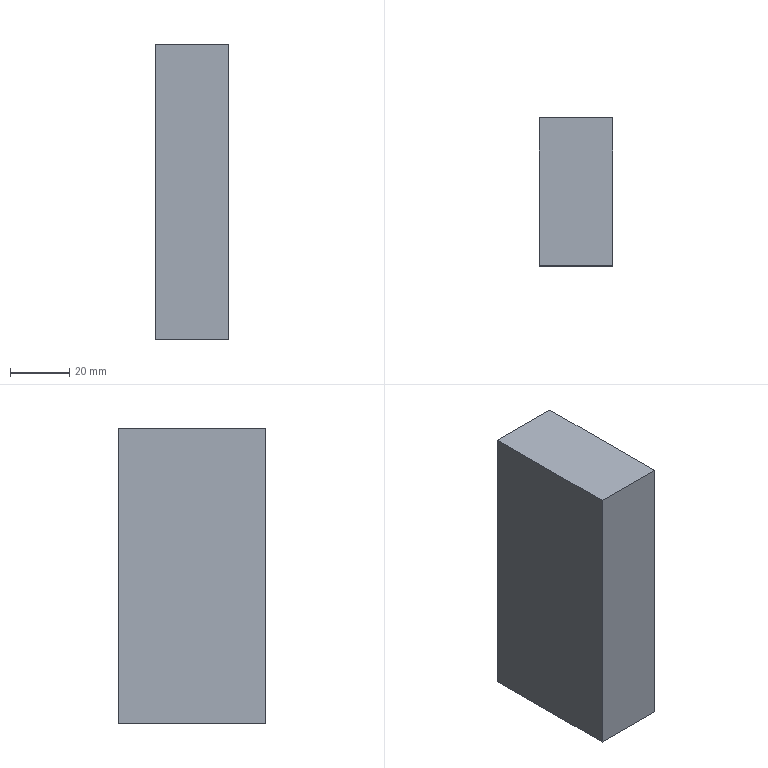Component | NX | SIDE | 1 solid | 6 faces | box 25 x 50 x 100 mm | volume 125000 mm3 | plane 6
STEP:
#1=CARTESIAN_POINT('',(0.,0.,0.));
#2=DIRECTION('',(0.,0.,1.));
#3=DIRECTION('',(1.,0.,0.));
#4=AXIS2_PLACEMENT_3D('',#1,#2,#3);
#5=CARTESIAN_POINT('',(530.662,30.,80.));
#6=VERTEX_POINT('',#5);
#7=CARTESIAN_POINT('',(530.662,30.,-20.));
#8=VERTEX_POINT('',#7);
#9=CARTESIAN_POINT('',(530.662,30.,80.));
#10=DIRECTION('',(0.,-0.,-1.));
#11=VECTOR('',#10,1.);
#12=LINE('',#9,#11);
#13=CARTESIAN_POINT('',(505.662,30.,80.));
#14=DIRECTION('',(0.,-1.,0.));
#15=DIRECTION('',(0.,-0.,-1.));
#16=AXIS2_PLACEMENT_3D('',#13,#14,#15);
#17=PLANE('',#16);
#18=CARTESIAN_POINT('',(0.,25.));
#19=DIRECTION('',(1.,0.));
#20=VECTOR('',#19,1.);
#21=LINE('',#18,#20);
#22=(GEOMETRIC_REPRESENTATION_CONTEXT(2)PARAMETRIC_REPRESENTATION_CONTEXT()REPRESENTATION_CONTEXT('',''));
#23=DEFINITIONAL_REPRESENTATION('',(#21),#22);
#24=PCURVE('',#17,#23);
#25=CARTESIAN_POINT('',(530.662,30.,-20.));
#26=DIRECTION('',(-1.,0.,0.));
#27=DIRECTION('',(0.,0.,-1.));
#28=AXIS2_PLACEMENT_3D('',#25,#26,#27);
#29=PLANE('',#28);
#30=CARTESIAN_POINT('',(-100.,0.));
#31=DIRECTION('',(1.,0.));
#32=VECTOR('',#31,1.);
#33=LINE('',#30,#32);
#34=(GEOMETRIC_REPRESENTATION_CONTEXT(2)PARAMETRIC_REPRESENTATION_CONTEXT()REPRESENTATION_CONTEXT('',''));
#35=DEFINITIONAL_REPRESENTATION('',(#33),#34);
#36=PCURVE('',#29,#35);
#37=SURFACE_CURVE('',#12,(#24,#36),.PCURVE_S1.);
#38=EDGE_CURVE('',#6,#8,#37,.T.);
#39=ORIENTED_EDGE('',*,*,#38,.T.);
#40=CARTESIAN_POINT('',(505.662,30.,-20.));
#41=VERTEX_POINT('',#40);
#42=CARTESIAN_POINT('',(505.662,30.,-20.));
#43=DIRECTION('',(1.,0.,0.));
#44=VECTOR('',#43,1.);
#45=LINE('',#42,#44);
#46=CARTESIAN_POINT('',(100.,0.));
#47=DIRECTION('',(0.,1.));
#48=VECTOR('',#47,1.);
#49=LINE('',#46,#48);
#50=(GEOMETRIC_REPRESENTATION_CONTEXT(2)PARAMETRIC_REPRESENTATION_CONTEXT()REPRESENTATION_CONTEXT('',''));
#51=DEFINITIONAL_REPRESENTATION('',(#49),#50);
#52=PCURVE('',#17,#51);
#53=CARTESIAN_POINT('',(505.662,30.,-20.));
#54=DIRECTION('',(0.,0.,1.));
#55=DIRECTION('',(0.,-1.,0.));
#56=AXIS2_PLACEMENT_3D('',#53,#54,#55);
#57=PLANE('',#56);
#58=CARTESIAN_POINT('',(0.,0.));
#59=DIRECTION('',(0.,1.));
#60=VECTOR('',#59,1.);
#61=LINE('',#58,#60);
#62=(GEOMETRIC_REPRESENTATION_CONTEXT(2)PARAMETRIC_REPRESENTATION_CONTEXT()REPRESENTATION_CONTEXT('',''));
#63=DEFINITIONAL_REPRESENTATION('',(#61),#62);
#64=PCURVE('',#57,#63);
#65=SURFACE_CURVE('',#45,(#52,#64),.PCURVE_S1.);
#66=EDGE_CURVE('',#41,#8,#65,.T.);
#67=ORIENTED_EDGE('',*,*,#66,.F.);
#68=CARTESIAN_POINT('',(505.662,30.,80.));
#69=VERTEX_POINT('',#68);
#70=CARTESIAN_POINT('',(505.662,30.,80.));
#71=DIRECTION('',(0.,-0.,-1.));
#72=VECTOR('',#71,1.);
#73=LINE('',#70,#72);
#74=CARTESIAN_POINT('',(0.,0.));
#75=DIRECTION('',(1.,0.));
#76=VECTOR('',#75,1.);
#77=LINE('',#74,#76);
#78=(GEOMETRIC_REPRESENTATION_CONTEXT(2)PARAMETRIC_REPRESENTATION_CONTEXT()REPRESENTATION_CONTEXT('',''));
#79=DEFINITIONAL_REPRESENTATION('',(#77),#78);
#80=PCURVE('',#17,#79);
#81=CARTESIAN_POINT('',(505.662,30.,-20.));
#82=DIRECTION('',(-1.,0.,0.));
#83=DIRECTION('',(0.,0.,-1.));
#84=AXIS2_PLACEMENT_3D('',#81,#82,#83);
#85=PLANE('',#84);
#86=CARTESIAN_POINT('',(-100.,0.));
#87=DIRECTION('',(1.,0.));
#88=VECTOR('',#87,1.);
#89=LINE('',#86,#88);
#90=(GEOMETRIC_REPRESENTATION_CONTEXT(2)PARAMETRIC_REPRESENTATION_CONTEXT()REPRESENTATION_CONTEXT('',''));
#91=DEFINITIONAL_REPRESENTATION('',(#89),#90);
#92=PCURVE('',#85,#91);
#93=SURFACE_CURVE('',#73,(#80,#92),.PCURVE_S1.);
#94=EDGE_CURVE('',#69,#41,#93,.T.);
#95=ORIENTED_EDGE('',*,*,#94,.F.);
#96=CARTESIAN_POINT('',(505.662,30.,80.));
#97=DIRECTION('',(1.,0.,0.));
#98=VECTOR('',#97,1.);
#99=LINE('',#96,#98);
#100=CARTESIAN_POINT('',(0.,0.));
#101=DIRECTION('',(0.,1.));
#102=VECTOR('',#101,1.);
#103=LINE('',#100,#102);
#104=(GEOMETRIC_REPRESENTATION_CONTEXT(2)PARAMETRIC_REPRESENTATION_CONTEXT()REPRESENTATION_CONTEXT('',''));
#105=DEFINITIONAL_REPRESENTATION('',(#103),#104);
#106=PCURVE('',#17,#105);
#107=CARTESIAN_POINT('',(505.662,-20.,80.));
#108=DIRECTION('',(0.,0.,-1.));
#109=DIRECTION('',(0.,1.,0.));
#110=AXIS2_PLACEMENT_3D('',#107,#108,#109);
#111=PLANE('',#110);
#112=CARTESIAN_POINT('',(50.,0.));
#113=DIRECTION('',(0.,1.));
#114=VECTOR('',#113,1.);
#115=LINE('',#112,#114);
#116=(GEOMETRIC_REPRESENTATION_CONTEXT(2)PARAMETRIC_REPRESENTATION_CONTEXT()REPRESENTATION_CONTEXT('',''));
#117=DEFINITIONAL_REPRESENTATION('',(#115),#116);
#118=PCURVE('',#111,#117);
#119=SURFACE_CURVE('',#99,(#106,#118),.PCURVE_S1.);
#120=EDGE_CURVE('',#69,#6,#119,.T.);
#121=ORIENTED_EDGE('',*,*,#120,.T.);
#122=EDGE_LOOP('',(#39,#67,#95,#121));
#123=FACE_BOUND('',#122,.T.);
#124=ADVANCED_FACE('',(#123),#17,.F.);
#125=CARTESIAN_POINT('',(530.662,-20.,-20.));
#126=VERTEX_POINT('',#125);
#127=CARTESIAN_POINT('',(530.662,30.,-20.));
#128=DIRECTION('',(0.,-1.,0.));
#129=VECTOR('',#128,1.);
#130=LINE('',#127,#129);
#131=CARTESIAN_POINT('',(0.,25.));
#132=DIRECTION('',(1.,0.));
#133=VECTOR('',#132,1.);
#134=LINE('',#131,#133);
#135=(GEOMETRIC_REPRESENTATION_CONTEXT(2)PARAMETRIC_REPRESENTATION_CONTEXT()REPRESENTATION_CONTEXT('',''));
#136=DEFINITIONAL_REPRESENTATION('',(#134),#135);
#137=PCURVE('',#57,#136);
#138=CARTESIAN_POINT('',(0.,0.));
#139=DIRECTION('',(0.,1.));
#140=VECTOR('',#139,1.);
#141=LINE('',#138,#140);
#142=(GEOMETRIC_REPRESENTATION_CONTEXT(2)PARAMETRIC_REPRESENTATION_CONTEXT()REPRESENTATION_CONTEXT('',''));
#143=DEFINITIONAL_REPRESENTATION('',(#141),#142);
#144=PCURVE('',#29,#143);
#145=SURFACE_CURVE('',#130,(#137,#144),.PCURVE_S1.);
#146=EDGE_CURVE('',#8,#126,#145,.T.);
#147=ORIENTED_EDGE('',*,*,#146,.T.);
#148=CARTESIAN_POINT('',(505.662,-20.,-20.));
#149=VERTEX_POINT('',#148);
#150=CARTESIAN_POINT('',(505.662,-20.,-20.));
#151=DIRECTION('',(1.,0.,0.));
#152=VECTOR('',#151,1.);
#153=LINE('',#150,#152);
#154=CARTESIAN_POINT('',(50.,0.));
#155=DIRECTION('',(0.,1.));
#156=VECTOR('',#155,1.);
#157=LINE('',#154,#156);
#158=(GEOMETRIC_REPRESENTATION_CONTEXT(2)PARAMETRIC_REPRESENTATION_CONTEXT()REPRESENTATION_CONTEXT('',''));
#159=DEFINITIONAL_REPRESENTATION('',(#157),#158);
#160=PCURVE('',#57,#159);
#161=CARTESIAN_POINT('',(505.662,-20.,-20.));
#162=DIRECTION('',(0.,1.,-0.));
#163=DIRECTION('',(0.,0.,1.));
#164=AXIS2_PLACEMENT_3D('',#161,#162,#163);
#165=PLANE('',#164);
#166=CARTESIAN_POINT('',(0.,0.));
#167=DIRECTION('',(0.,1.));
#168=VECTOR('',#167,1.);
#169=LINE('',#166,#168);
#170=(GEOMETRIC_REPRESENTATION_CONTEXT(2)PARAMETRIC_REPRESENTATION_CONTEXT()REPRESENTATION_CONTEXT('',''));
#171=DEFINITIONAL_REPRESENTATION('',(#169),#170);
#172=PCURVE('',#165,#171);
#173=SURFACE_CURVE('',#153,(#160,#172),.PCURVE_S1.);
#174=EDGE_CURVE('',#149,#126,#173,.T.);
#175=ORIENTED_EDGE('',*,*,#174,.F.);
#176=CARTESIAN_POINT('',(505.662,30.,-20.));
#177=DIRECTION('',(0.,-1.,0.));
#178=VECTOR('',#177,1.);
#179=LINE('',#176,#178);
#180=CARTESIAN_POINT('',(0.,0.));
#181=DIRECTION('',(1.,0.));
#182=VECTOR('',#181,1.);
#183=LINE('',#180,#182);
#184=(GEOMETRIC_REPRESENTATION_CONTEXT(2)PARAMETRIC_REPRESENTATION_CONTEXT()REPRESENTATION_CONTEXT('',''));
#185=DEFINITIONAL_REPRESENTATION('',(#183),#184);
#186=PCURVE('',#57,#185);
#187=CARTESIAN_POINT('',(0.,0.));
#188=DIRECTION('',(0.,1.));
#189=VECTOR('',#188,1.);
#190=LINE('',#187,#189);
#191=(GEOMETRIC_REPRESENTATION_CONTEXT(2)PARAMETRIC_REPRESENTATION_CONTEXT()REPRESENTATION_CONTEXT('',''));
#192=DEFINITIONAL_REPRESENTATION('',(#190),#191);
#193=PCURVE('',#85,#192);
#194=SURFACE_CURVE('',#179,(#186,#193),.PCURVE_S1.);
#195=EDGE_CURVE('',#41,#149,#194,.T.);
#196=ORIENTED_EDGE('',*,*,#195,.F.);
#197=ORIENTED_EDGE('',*,*,#66,.T.);
#198=EDGE_LOOP('',(#147,#175,#196,#197));
#199=FACE_BOUND('',#198,.T.);
#200=ADVANCED_FACE('',(#199),#57,.F.);
#201=CARTESIAN_POINT('',(530.662,-20.,80.));
#202=VERTEX_POINT('',#201);
#203=CARTESIAN_POINT('',(530.662,-20.,-20.));
#204=DIRECTION('',(0.,0.,1.));
#205=VECTOR('',#204,1.);
#206=LINE('',#203,#205);
#207=CARTESIAN_POINT('',(0.,25.));
#208=DIRECTION('',(1.,0.));
#209=VECTOR('',#208,1.);
#210=LINE('',#207,#209);
#211=(GEOMETRIC_REPRESENTATION_CONTEXT(2)PARAMETRIC_REPRESENTATION_CONTEXT()REPRESENTATION_CONTEXT('',''));
#212=DEFINITIONAL_REPRESENTATION('',(#210),#211);
#213=PCURVE('',#165,#212);
#214=CARTESIAN_POINT('',(0.,50.));
#215=DIRECTION('',(-1.,-0.));
#216=VECTOR('',#215,1.);
#217=LINE('',#214,#216);
#218=(GEOMETRIC_REPRESENTATION_CONTEXT(2)PARAMETRIC_REPRESENTATION_CONTEXT()REPRESENTATION_CONTEXT('',''));
#219=DEFINITIONAL_REPRESENTATION('',(#217),#218);
#220=PCURVE('',#29,#219);
#221=SURFACE_CURVE('',#206,(#213,#220),.PCURVE_S1.);
#222=EDGE_CURVE('',#126,#202,#221,.T.);
#223=ORIENTED_EDGE('',*,*,#222,.T.);
#224=CARTESIAN_POINT('',(505.662,-20.,80.));
#225=VERTEX_POINT('',#224);
#226=CARTESIAN_POINT('',(505.662,-20.,80.));
#227=DIRECTION('',(1.,0.,0.));
#228=VECTOR('',#227,1.);
#229=LINE('',#226,#228);
#230=CARTESIAN_POINT('',(100.,0.));
#231=DIRECTION('',(0.,1.));
#232=VECTOR('',#231,1.);
#233=LINE('',#230,#232);
#234=(GEOMETRIC_REPRESENTATION_CONTEXT(2)PARAMETRIC_REPRESENTATION_CONTEXT()REPRESENTATION_CONTEXT('',''));
#235=DEFINITIONAL_REPRESENTATION('',(#233),#234);
#236=PCURVE('',#165,#235);
#237=CARTESIAN_POINT('',(0.,0.));
#238=DIRECTION('',(0.,1.));
#239=VECTOR('',#238,1.);
#240=LINE('',#237,#239);
#241=(GEOMETRIC_REPRESENTATION_CONTEXT(2)PARAMETRIC_REPRESENTATION_CONTEXT()REPRESENTATION_CONTEXT('',''));
#242=DEFINITIONAL_REPRESENTATION('',(#240),#241);
#243=PCURVE('',#111,#242);
#244=SURFACE_CURVE('',#229,(#236,#243),.PCURVE_S1.);
#245=EDGE_CURVE('',#225,#202,#244,.T.);
#246=ORIENTED_EDGE('',*,*,#245,.F.);
#247=CARTESIAN_POINT('',(505.662,-20.,-20.));
#248=DIRECTION('',(0.,0.,1.));
#249=VECTOR('',#248,1.);
#250=LINE('',#247,#249);
#251=CARTESIAN_POINT('',(0.,0.));
#252=DIRECTION('',(1.,0.));
#253=VECTOR('',#252,1.);
#254=LINE('',#251,#253);
#255=(GEOMETRIC_REPRESENTATION_CONTEXT(2)PARAMETRIC_REPRESENTATION_CONTEXT()REPRESENTATION_CONTEXT('',''));
#256=DEFINITIONAL_REPRESENTATION('',(#254),#255);
#257=PCURVE('',#165,#256);
#258=CARTESIAN_POINT('',(0.,50.));
#259=DIRECTION('',(-1.,-0.));
#260=VECTOR('',#259,1.);
#261=LINE('',#258,#260);
#262=(GEOMETRIC_REPRESENTATION_CONTEXT(2)PARAMETRIC_REPRESENTATION_CONTEXT()REPRESENTATION_CONTEXT('',''));
#263=DEFINITIONAL_REPRESENTATION('',(#261),#262);
#264=PCURVE('',#85,#263);
#265=SURFACE_CURVE('',#250,(#257,#264),.PCURVE_S1.);
#266=EDGE_CURVE('',#149,#225,#265,.T.);
#267=ORIENTED_EDGE('',*,*,#266,.F.);
#268=ORIENTED_EDGE('',*,*,#174,.T.);
#269=EDGE_LOOP('',(#223,#246,#267,#268));
#270=FACE_BOUND('',#269,.T.);
#271=ADVANCED_FACE('',(#270),#165,.F.);
#272=CARTESIAN_POINT('',(530.662,-20.,80.));
#273=DIRECTION('',(0.,1.,0.));
#274=VECTOR('',#273,1.);
#275=LINE('',#272,#274);
#276=CARTESIAN_POINT('',(0.,25.));
#277=DIRECTION('',(1.,0.));
#278=VECTOR('',#277,1.);
#279=LINE('',#276,#278);
#280=(GEOMETRIC_REPRESENTATION_CONTEXT(2)PARAMETRIC_REPRESENTATION_CONTEXT()REPRESENTATION_CONTEXT('',''));
#281=DEFINITIONAL_REPRESENTATION('',(#279),#280);
#282=PCURVE('',#111,#281);
#283=CARTESIAN_POINT('',(-100.,50.));
#284=DIRECTION('',(0.,-1.));
#285=VECTOR('',#284,1.);
#286=LINE('',#283,#285);
#287=(GEOMETRIC_REPRESENTATION_CONTEXT(2)PARAMETRIC_REPRESENTATION_CONTEXT()REPRESENTATION_CONTEXT('',''));
#288=DEFINITIONAL_REPRESENTATION('',(#286),#287);
#289=PCURVE('',#29,#288);
#290=SURFACE_CURVE('',#275,(#282,#289),.PCURVE_S1.);
#291=EDGE_CURVE('',#202,#6,#290,.T.);
#292=ORIENTED_EDGE('',*,*,#291,.T.);
#293=ORIENTED_EDGE('',*,*,#120,.F.);
#294=CARTESIAN_POINT('',(505.662,-20.,80.));
#295=DIRECTION('',(0.,1.,0.));
#296=VECTOR('',#295,1.);
#297=LINE('',#294,#296);
#298=CARTESIAN_POINT('',(0.,0.));
#299=DIRECTION('',(1.,0.));
#300=VECTOR('',#299,1.);
#301=LINE('',#298,#300);
#302=(GEOMETRIC_REPRESENTATION_CONTEXT(2)PARAMETRIC_REPRESENTATION_CONTEXT()REPRESENTATION_CONTEXT('',''));
#303=DEFINITIONAL_REPRESENTATION('',(#301),#302);
#304=PCURVE('',#111,#303);
#305=CARTESIAN_POINT('',(-100.,50.));
#306=DIRECTION('',(0.,-1.));
#307=VECTOR('',#306,1.);
#308=LINE('',#305,#307);
#309=(GEOMETRIC_REPRESENTATION_CONTEXT(2)PARAMETRIC_REPRESENTATION_CONTEXT()REPRESENTATION_CONTEXT('',''));
#310=DEFINITIONAL_REPRESENTATION('',(#308),#309);
#311=PCURVE('',#85,#310);
#312=SURFACE_CURVE('',#297,(#304,#311),.PCURVE_S1.);
#313=EDGE_CURVE('',#225,#69,#312,.T.);
#314=ORIENTED_EDGE('',*,*,#313,.F.);
#315=ORIENTED_EDGE('',*,*,#245,.T.);
#316=EDGE_LOOP('',(#292,#293,#314,#315));
#317=FACE_BOUND('',#316,.T.);
#318=ADVANCED_FACE('',(#317),#111,.F.);
#319=ORIENTED_EDGE('',*,*,#94,.T.);
#320=ORIENTED_EDGE('',*,*,#195,.T.);
#321=ORIENTED_EDGE('',*,*,#266,.T.);
#322=ORIENTED_EDGE('',*,*,#313,.T.);
#323=EDGE_LOOP('',(#319,#320,#321,#322));
#324=FACE_BOUND('',#323,.T.);
#325=ADVANCED_FACE('',(#324),#85,.T.);
#326=ORIENTED_EDGE('',*,*,#38,.F.);
#327=ORIENTED_EDGE('',*,*,#291,.F.);
#328=ORIENTED_EDGE('',*,*,#222,.F.);
#329=ORIENTED_EDGE('',*,*,#146,.F.);
#330=EDGE_LOOP('',(#326,#327,#328,#329));
#331=FACE_BOUND('',#330,.T.);
#332=ADVANCED_FACE('',(#331),#29,.F.);
#333=CLOSED_SHELL('',(#124,#200,#271,#318,#325,#332));
#334=MANIFOLD_SOLID_BREP('',#333);
#335=(LENGTH_UNIT()NAMED_UNIT(*)SI_UNIT(.MILLI.,.METRE.));
#336=UNCERTAINTY_MEASURE_WITH_UNIT(LENGTH_MEASURE(0.0000001),#335,'','');
#337=(NAMED_UNIT(*)PLANE_ANGLE_UNIT()SI_UNIT($,.RADIAN.));
#338=(NAMED_UNIT(*)SI_UNIT($,.STERADIAN.)SOLID_ANGLE_UNIT());
#339=(GEOMETRIC_REPRESENTATION_CONTEXT(3)GLOBAL_UNCERTAINTY_ASSIGNED_CONTEXT((#336))GLOBAL_UNIT_ASSIGNED_CONTEXT((#335,#337,#338))REPRESENTATION_CONTEXT('',''));
#340=ADVANCED_BREP_SHAPE_REPRESENTATION('',(#4,#334),#339);